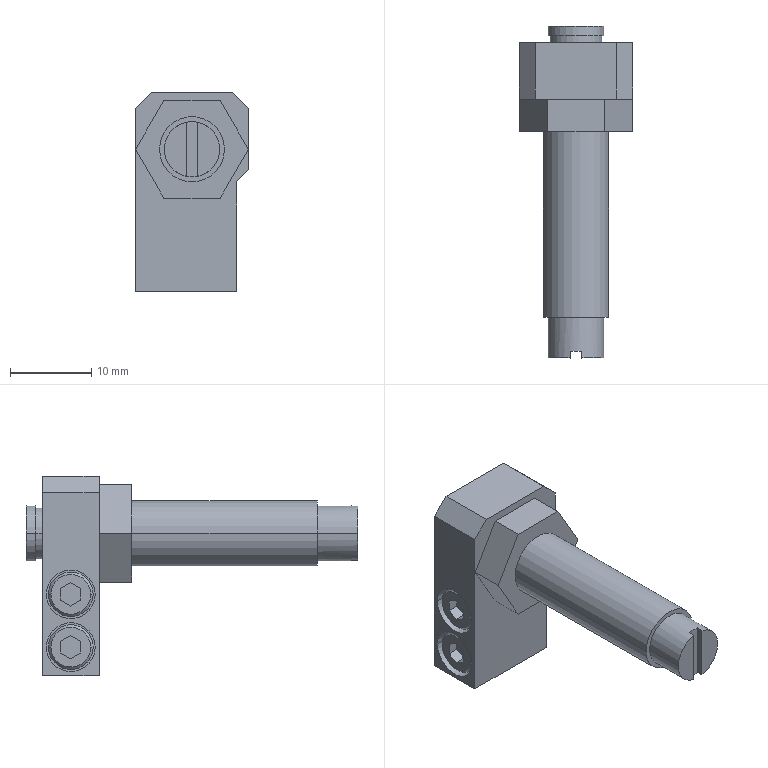Component | SolidWorks | MXQ8-30B-M9N_0_0_MXQ8-30B-M9N_0_0-2_MXQ8-30B-M9N_0_0_5_16-1 | 1 solid | 66 faces | volume 4048 mm3 | plane 44 | cylinder 18 | cone 4 | commonest cylinder face diameters 6.8 x4 6 x4 5.5 x4 8 x2 6.3 x2 2.8 x2